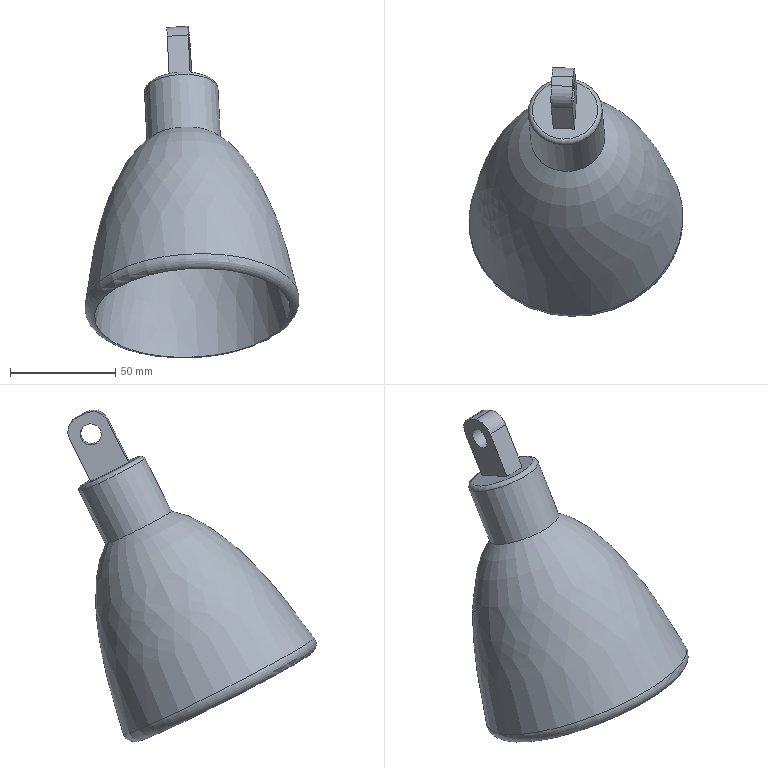Component | NX | REFLECTOR | 1 solid | 17 faces | volume 132447 mm3 | plane 7 | cylinder 6 | other 2 | torus 2 | commonest cylinder face diameters 15 x2 25 x1 35 x1 10 x1 4 x1